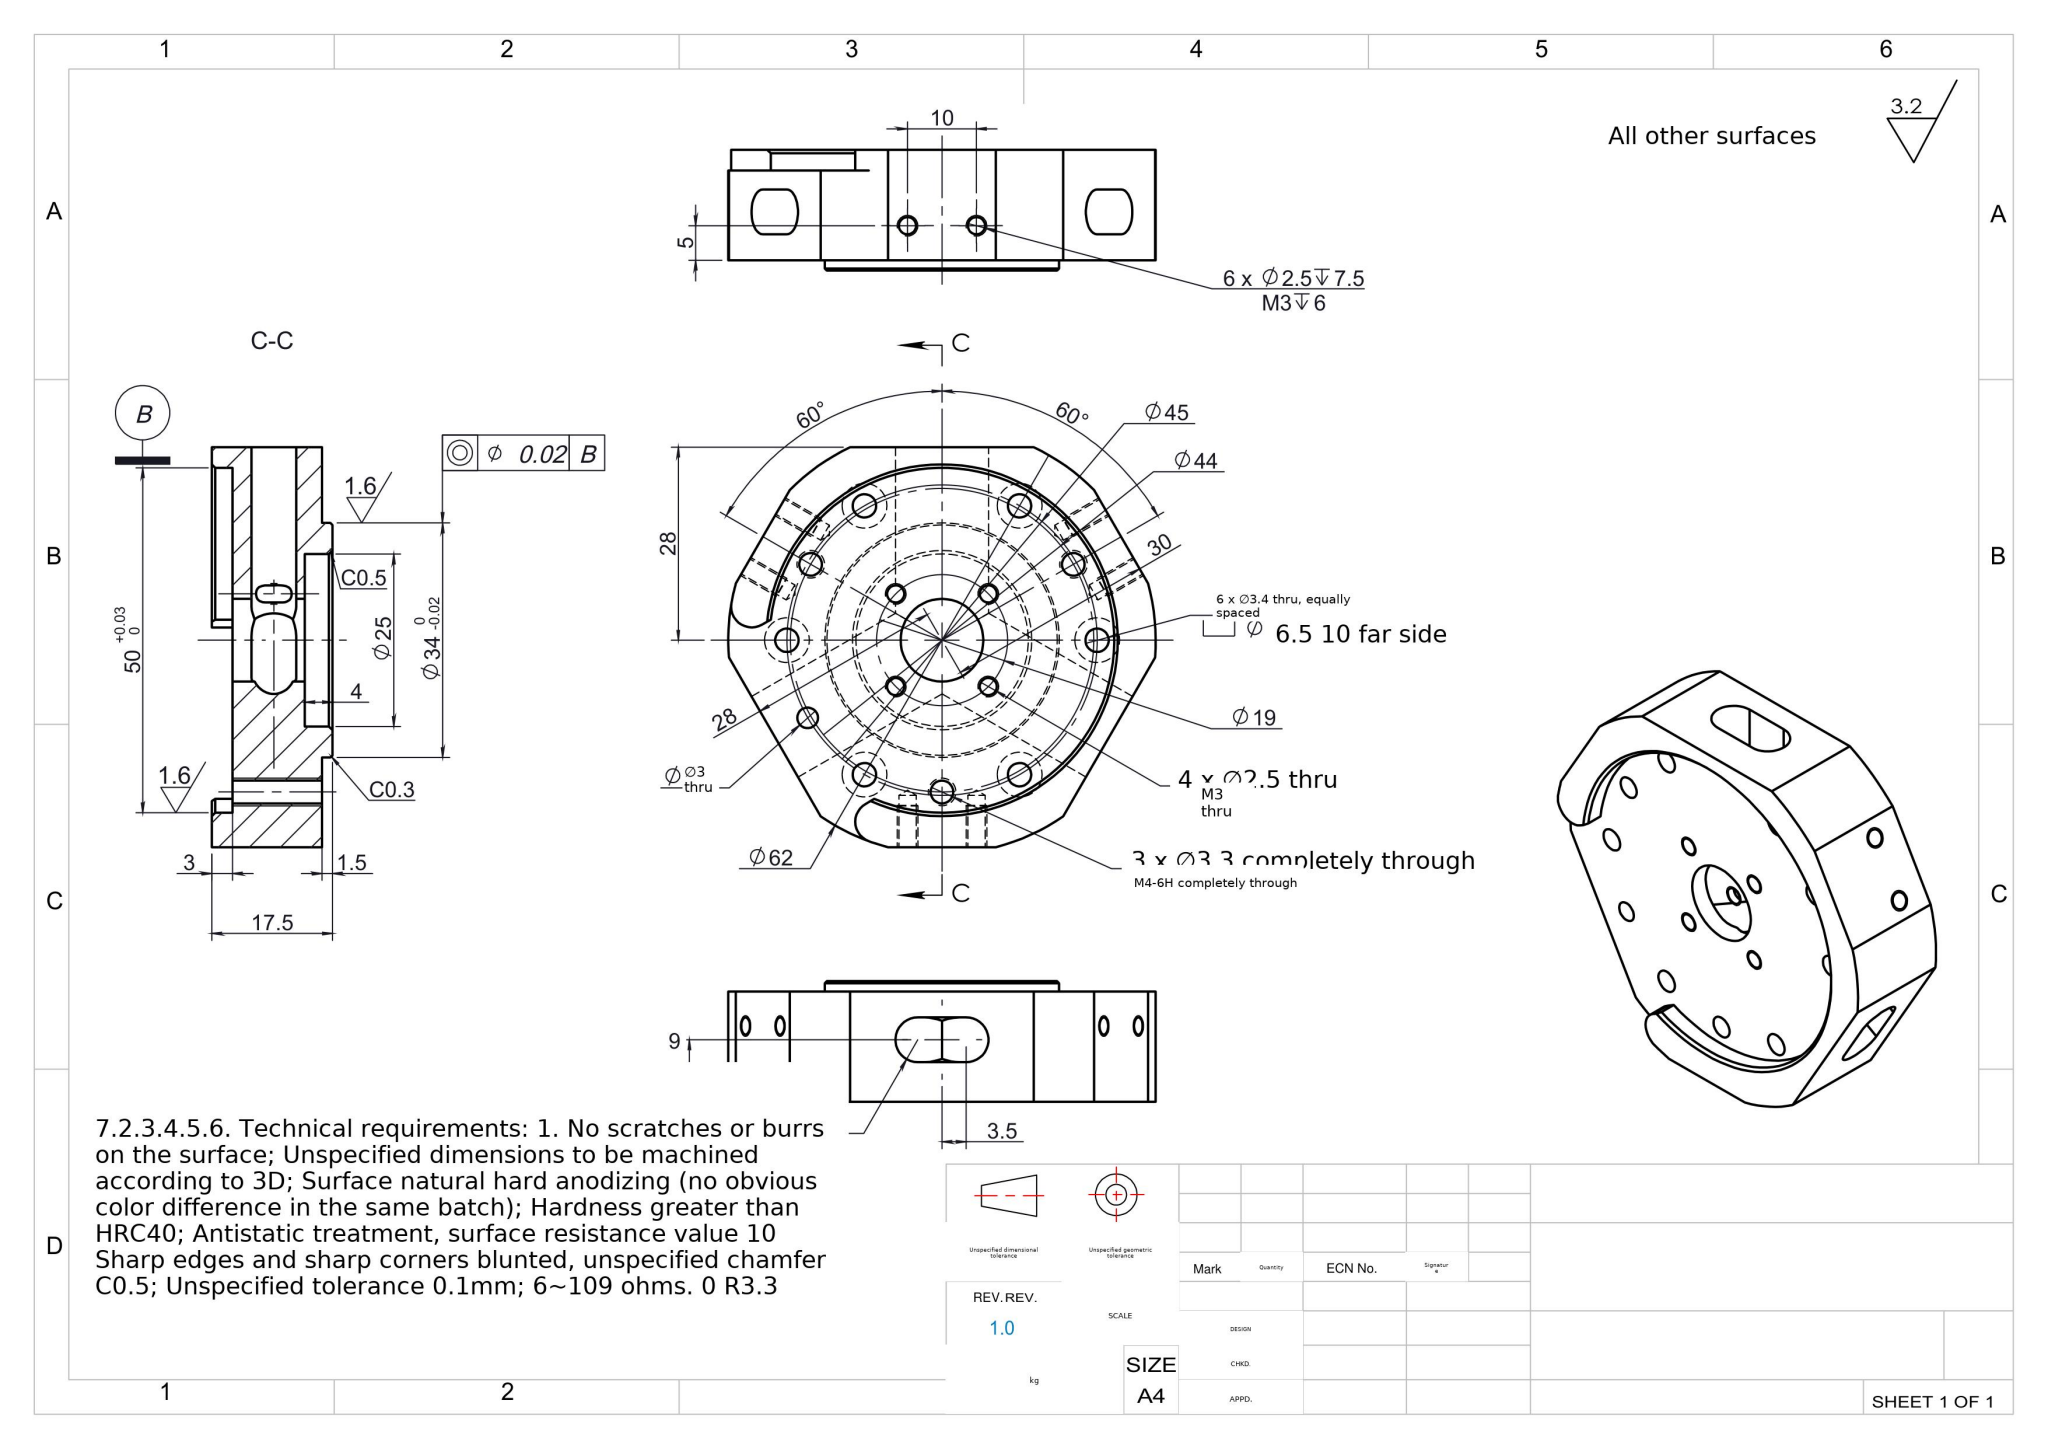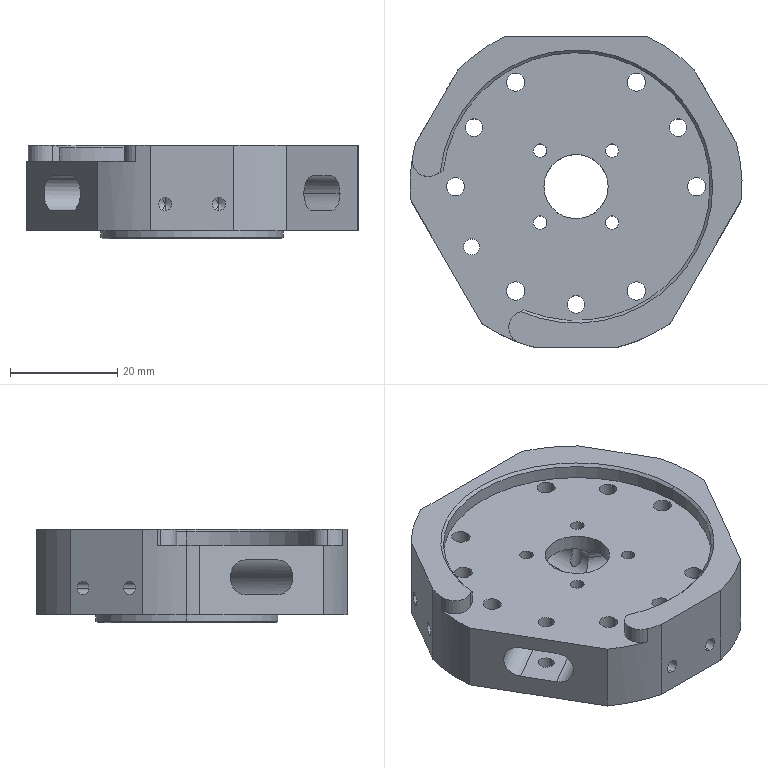Part | SolidWorks | mm | 1 solid | 131 faces | box 62 x 58 x 17.5 mm | volume 28711 mm3 | cylinder 88 | plane 25 | cone 18 | commonest cylinder face diameters 2.5 x24 6.5 x21 3.4 x12 62 x7 3.3 x6 12 x4 6 x4 3 x4